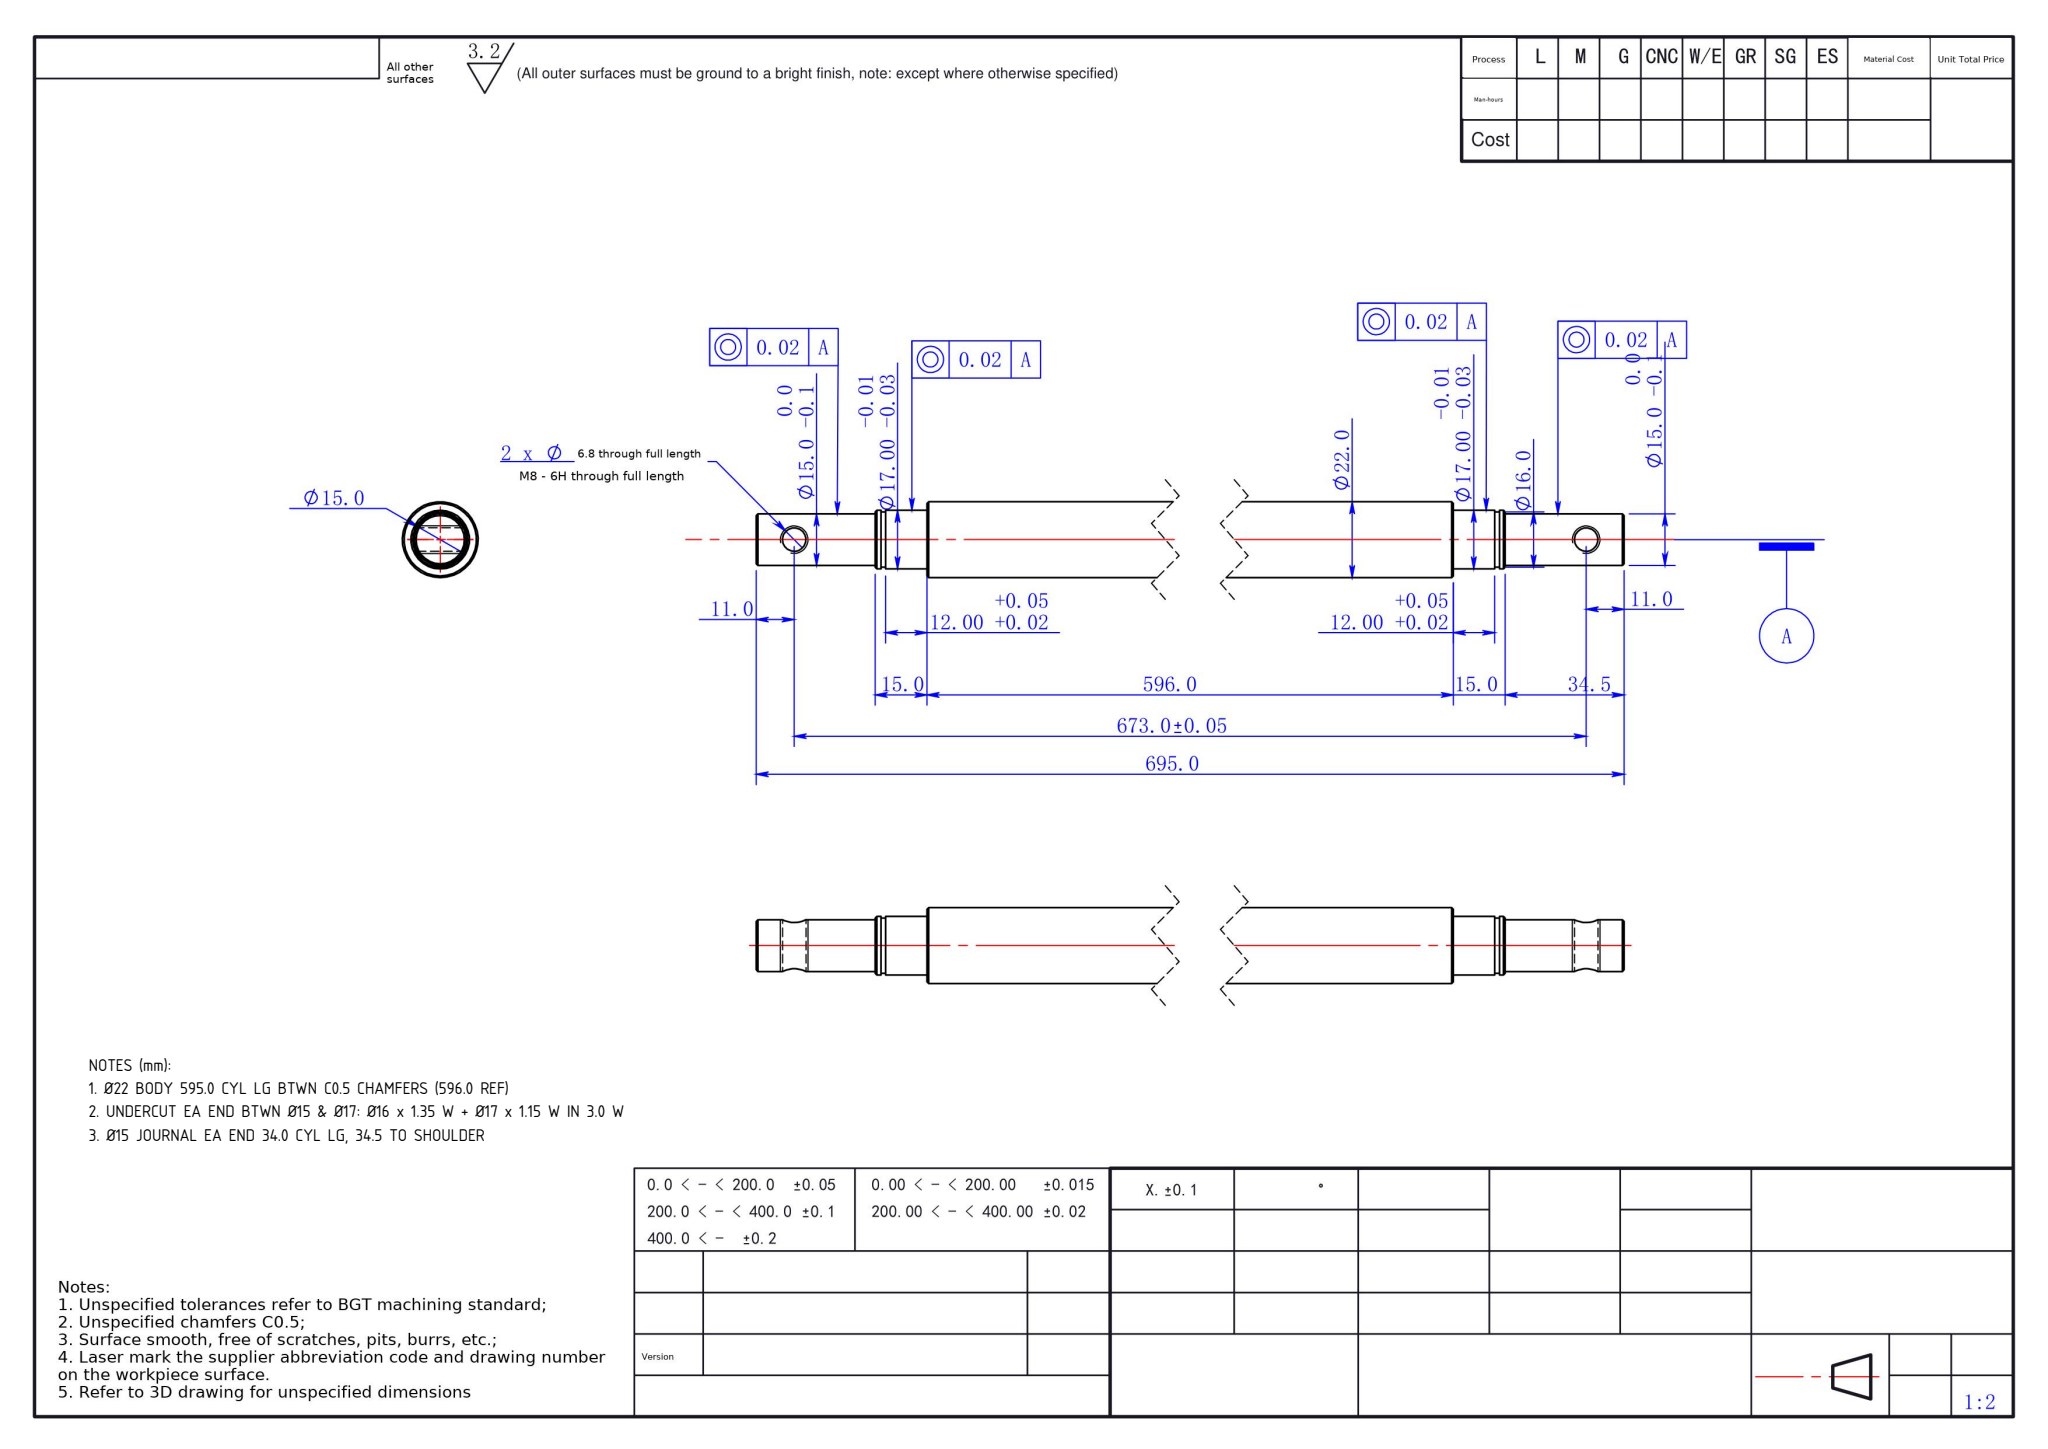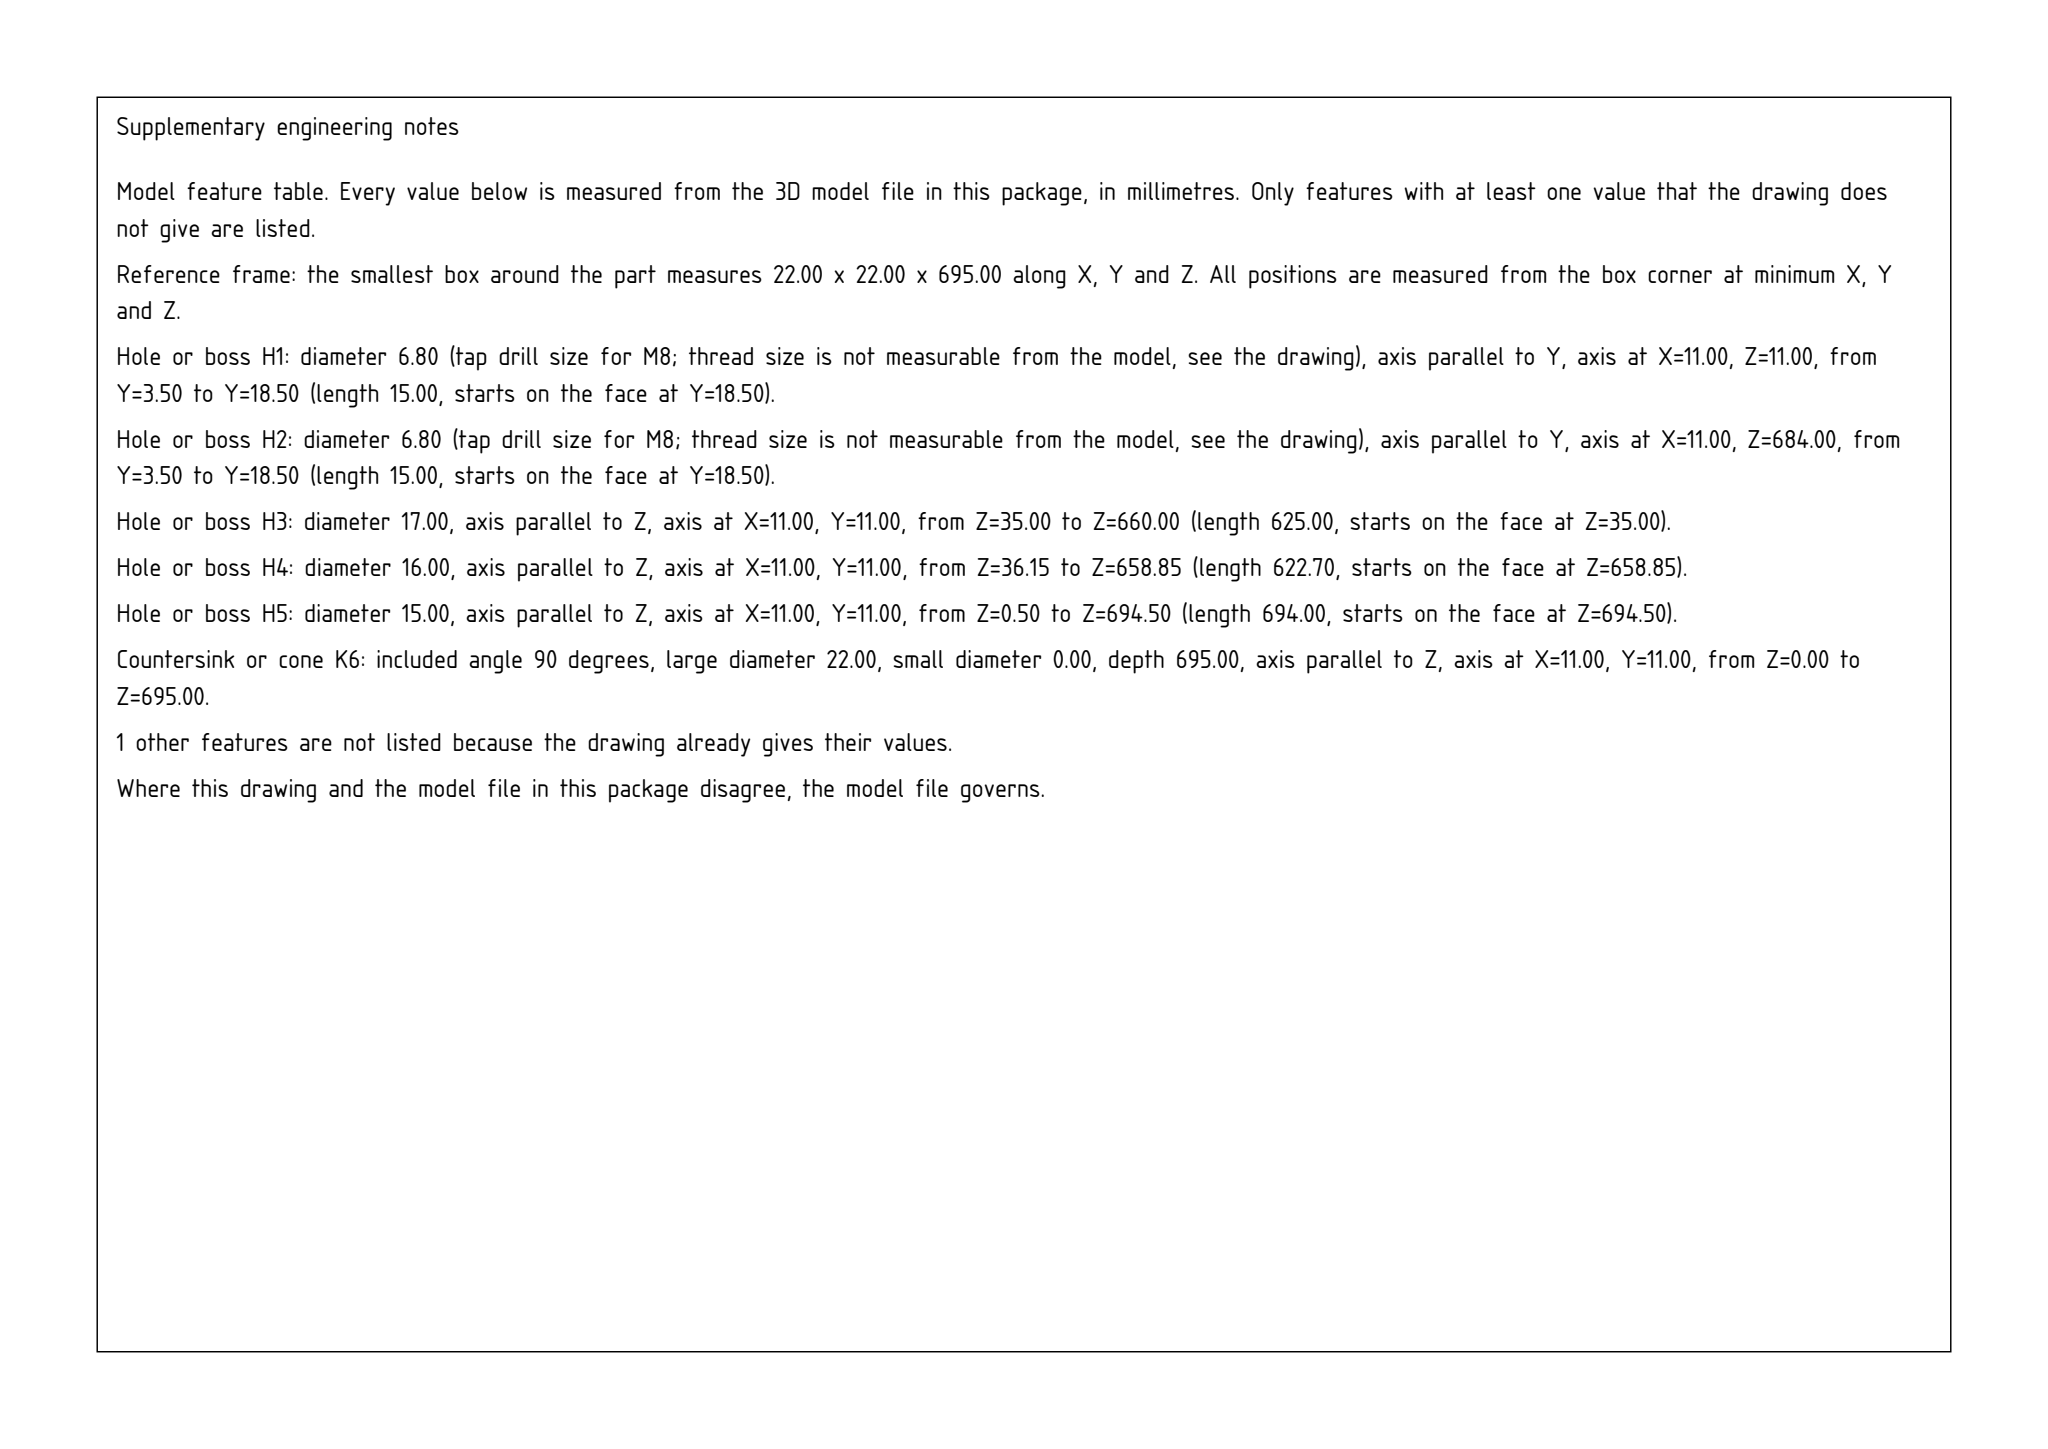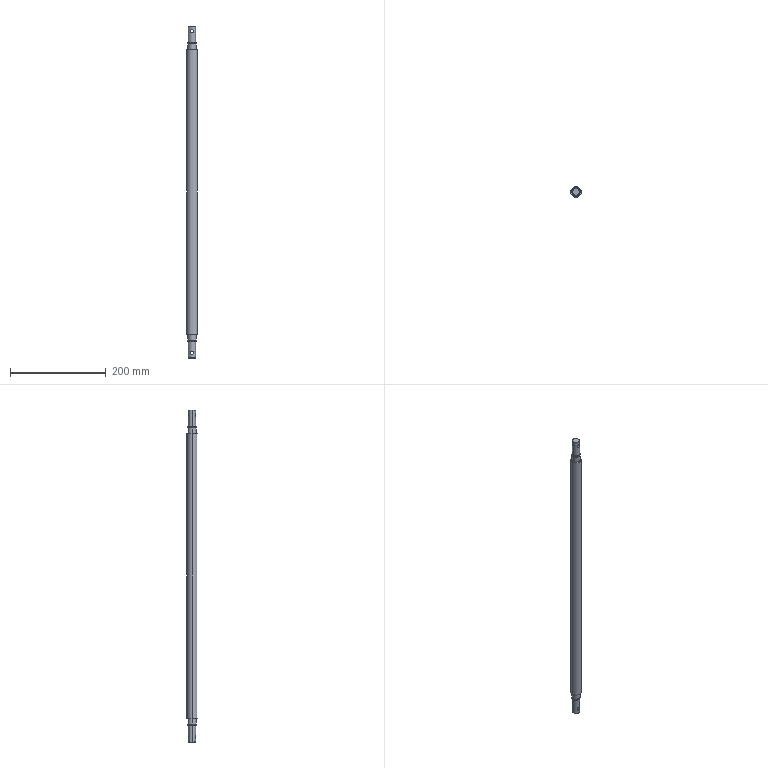Part | SolidWorks | mm | 1 solid | 44 faces | box 22 x 22 x 695 mm | volume 244389 mm3 | cylinder 22 | cone 12 | plane 10 | commonest cylinder face diameters 17 x8 6.8 x4 15 x4 16 x4 22 x2
Drawing notes:
Ø22 BODY 595.0 CYL LG BTWN C0.5 CHAMFERS (596.0 REF) | from the solid: Cylinder Ø22 z axis L=595.0; 90° cones ref Ø22/Ø21 at each end
UNDERCUT EA END BTWN Ø15 & Ø17: Ø16 x 1.35 W + Ø17 x 1.15 W IN 3.0 W | from the solid: Planes z=34.5/36.15/37.5 and z=657.5/658.85/660.5 give 3.0 gap; cyls Ø16 L=1.35, Ø17 L=1.15
Ø15 JOURNAL EA END 34.0 CYL LG, 34.5 TO SHOULDER | from the solid: Cylinder Ø15 z axis L=34.0; planes z=660.5/695.0 = 34.5; cone ref Ø15/Ø14 = C0.5 end chamfer
build123d program:
from build123d import *

# Parameters (mm, degrees)
CHAMFER1_SIZE     = 0.5
SKETCH4_W         = 0.5
SKETCH4_H         = 1.35
CHAMFER2_SIZE     = 0.5
M8_TAPPED_HOLE1_D = 6.8


with BuildPart() as part:
    # Sketch1 → Revolve1 (revolve)
    with BuildSketch(Plane(origin=(0, 0, 0), x_dir=(1, 0, 0), z_dir=(0, 1, 0))):
        Polygon((0, 0), (7.5, 0), (7.5, 34.5), (8.5, 34.5), (8.5, 49.5), (11, 49.5), (11, 645.5), (8.5, 645.5), (8.5, 660.5), (7.5, 660.5), (7.5, 695), (0, 695), align=None)
    revolve(axis=Axis((0, 0, 0), (0, 0, -1)))

    # Chamfer1
    chamfer1_edges = [part.edges().sort_by_distance(p)[0] for p in [
        (-7.5, 0, 0),
        (-7.5, 0, -695),
    ]]
    chamfer(chamfer1_edges, length=CHAMFER1_SIZE)

    # Sketch4 → Cut-Revolve1 (revolve, cut)
    with BuildSketch(Plane(origin=(0, 0, 0), x_dir=(1, 0, 0), z_dir=(0, 1, 0))):
        with Locations((8.25, 36.825)):
            Rectangle(SKETCH4_W, SKETCH4_H)
        with Locations((8.25, 658.175)):
            Rectangle(SKETCH4_W, SKETCH4_H)
    revolve(axis=Axis((0, 0, -34.5), (0, 0, -1)), mode=Mode.SUBTRACT)

    # Chamfer2
    chamfer2_edges = [part.edges().sort_by_distance(p)[0] for p in [
        (-11, 0, -645.5),
        (-11, 0, -49.5),
        (-8.5, 0, -34.5),
        (-8.5, 0, -660.5),
    ]]
    chamfer(chamfer2_edges, length=CHAMFER2_SIZE)

    # M8 Tapped Hole1 (through all)
    with Locations(Plane(origin=(0, 7.5, -11), x_dir=(1, 0, 0), z_dir=(0, 1, 0))):
        with Locations((0, 0), (0, 673)):
            Hole(M8_TAPPED_HOLE1_D / 2)


solid = part.part